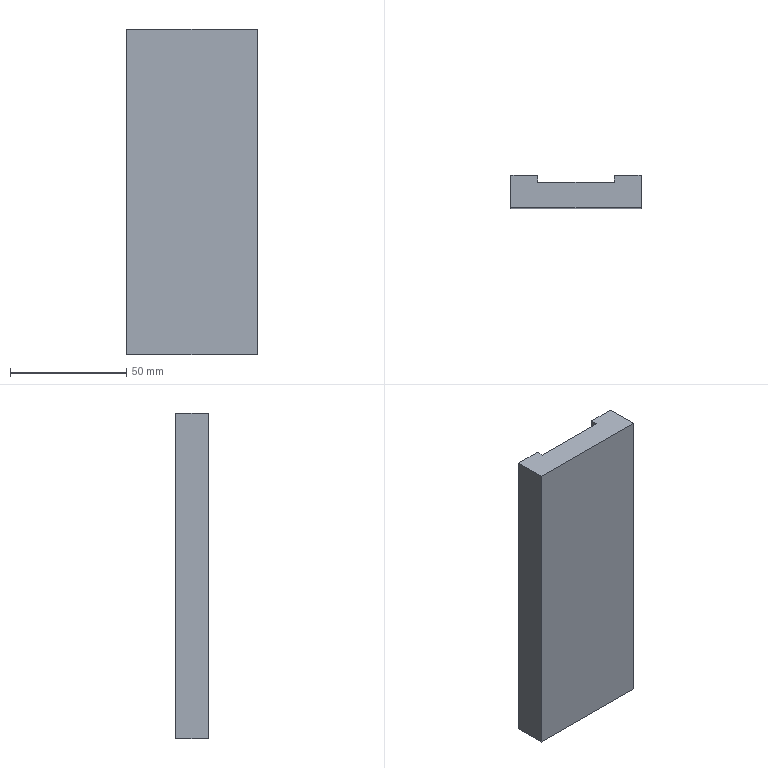Component | SolidWorks | CHEN123-AA-17-2 | 1 solid | 10 faces | box 56 x 14 x 140 mm | volume 95900 mm3 | plane 10
build123d program:
from build123d import *

# Parameters (mm, degrees)
SKETCH1_W           = 140
SKETCH1_H           = 56
BOSS_EXTRUDE1_DEPTH = 14
SKETCH3_W           = 197.23
SKETCH3_H           = 33
CUT_EXTRUDE2_DEPTH  = 3


with BuildPart() as part:
    # Sketch1 → Boss-Extrude1 (new body)
    with BuildSketch(Plane.XY):
        Rectangle(SKETCH1_W, SKETCH1_H)
    extrude(amount=BOSS_EXTRUDE1_DEPTH)

    # Sketch3 → Cut-Extrude2 (cut)
    with BuildSketch(Plane(origin=(0, 0, 0), x_dir=(-1, 0, 0), z_dir=(0, 0, -1))):
        Rectangle(SKETCH3_W, SKETCH3_H)
    extrude(amount=-CUT_EXTRUDE2_DEPTH, mode=Mode.SUBTRACT)


solid = part.part

# Placed as in the assembly
solid = solid.moved(Location((-0.0005, 34.001, -60), (90, 0, 90)))
STEP:
#1=CARTESIAN_POINT('',(-0.6496,1.339,-5.118));
#2=VERTEX_POINT('',#1);
#3=CARTESIAN_POINT('',(-0.6496,1.339,0.3937));
#4=VERTEX_POINT('',#3);
#5=CARTESIAN_POINT('',(-0.6496,1.339,-2.362));
#6=DIRECTION('',(0.,0.,1.));
#7=VECTOR('',#6,39.37);
#8=LINE('',#5,#7);
#9=EDGE_CURVE('',#2,#4,#8,.T.);
#10=ORIENTED_EDGE('',*,*,#9,.F.);
#11=CARTESIAN_POINT('',(-1.102,1.339,-5.118));
#12=VERTEX_POINT('',#11);
#13=CARTESIAN_POINT('',(1.102,1.339,-5.118));
#14=DIRECTION('',(1.,0.,-0.));
#15=VECTOR('',#14,39.37);
#16=LINE('',#13,#15);
#17=EDGE_CURVE('',#12,#2,#16,.T.);
#18=ORIENTED_EDGE('',*,*,#17,.F.);
#19=CARTESIAN_POINT('',(-1.102,1.339,0.3937));
#20=VERTEX_POINT('',#19);
#21=CARTESIAN_POINT('',(-1.102,1.339,-5.118));
#22=DIRECTION('',(-0.,0.,-1.));
#23=VECTOR('',#22,39.37);
#24=LINE('',#21,#23);
#25=EDGE_CURVE('',#20,#12,#24,.T.);
#26=ORIENTED_EDGE('',*,*,#25,.F.);
#27=CARTESIAN_POINT('',(1.102,1.339,0.3937));
#28=DIRECTION('',(-1.,0.,0.));
#29=VECTOR('',#28,39.37);
#30=LINE('',#27,#29);
#31=EDGE_CURVE('',#4,#20,#30,.T.);
#32=ORIENTED_EDGE('',*,*,#31,.F.);
#33=EDGE_LOOP('',(#10,#18,#26,#32));
#34=FACE_OUTER_BOUND('',#33,.T.);
#35=CARTESIAN_POINT('',(-0.00001969,1.339,-2.362));
#36=DIRECTION('',(0.,1.,0.));
#37=DIRECTION('',(-0.,0.,-1.));
#38=AXIS2_PLACEMENT_3D('',#35,#36,#37);
#39=PLANE('',#38);
#40=ADVANCED_FACE('',(#34),#39,.T.);
#41=CARTESIAN_POINT('',(0.6496,1.221,0.3937));
#42=VERTEX_POINT('',#41);
#43=CARTESIAN_POINT('',(-0.6496,1.221,0.3937));
#44=VERTEX_POINT('',#43);
#45=CARTESIAN_POINT('',(1.102,1.221,0.3937));
#46=DIRECTION('',(-1.,0.,0.));
#47=VECTOR('',#46,39.37);
#48=LINE('',#45,#47);
#49=EDGE_CURVE('',#42,#44,#48,.T.);
#50=ORIENTED_EDGE('',*,*,#49,.T.);
#51=CARTESIAN_POINT('',(-0.6496,0.7874,0.3937));
#52=DIRECTION('',(0.,1.,0.));
#53=VECTOR('',#52,39.37);
#54=LINE('',#51,#53);
#55=EDGE_CURVE('',#44,#4,#54,.T.);
#56=ORIENTED_EDGE('',*,*,#55,.T.);
#57=ORIENTED_EDGE('',*,*,#31,.T.);
#58=CARTESIAN_POINT('',(-1.102,0.7874,0.3937));
#59=VERTEX_POINT('',#58);
#60=CARTESIAN_POINT('',(-1.102,0.7874,0.3937));
#61=DIRECTION('',(0.,1.,0.));
#62=VECTOR('',#61,39.37);
#63=LINE('',#60,#62);
#64=EDGE_CURVE('',#59,#20,#63,.T.);
#65=ORIENTED_EDGE('',*,*,#64,.F.);
#66=CARTESIAN_POINT('',(1.102,0.7874,0.3937));
#67=VERTEX_POINT('',#66);
#68=CARTESIAN_POINT('',(1.102,0.7874,0.3937));
#69=DIRECTION('',(-1.,0.,0.));
#70=VECTOR('',#69,39.37);
#71=LINE('',#68,#70);
#72=EDGE_CURVE('',#67,#59,#71,.T.);
#73=ORIENTED_EDGE('',*,*,#72,.F.);
#74=CARTESIAN_POINT('',(1.102,1.339,0.3937));
#75=VERTEX_POINT('',#74);
#76=CARTESIAN_POINT('',(1.102,0.7874,0.3937));
#77=DIRECTION('',(0.,1.,0.));
#78=VECTOR('',#77,39.37);
#79=LINE('',#76,#78);
#80=EDGE_CURVE('',#67,#75,#79,.T.);
#81=ORIENTED_EDGE('',*,*,#80,.T.);
#82=CARTESIAN_POINT('',(0.6496,1.339,0.3937));
#83=VERTEX_POINT('',#82);
#84=CARTESIAN_POINT('',(1.102,1.339,0.3937));
#85=DIRECTION('',(-1.,0.,0.));
#86=VECTOR('',#85,39.37);
#87=LINE('',#84,#86);
#88=EDGE_CURVE('',#75,#83,#87,.T.);
#89=ORIENTED_EDGE('',*,*,#88,.T.);
#90=CARTESIAN_POINT('',(0.6496,0.7874,0.3937));
#91=DIRECTION('',(0.,-1.,0.));
#92=VECTOR('',#91,39.37);
#93=LINE('',#90,#92);
#94=EDGE_CURVE('',#83,#42,#93,.T.);
#95=ORIENTED_EDGE('',*,*,#94,.T.);
#96=EDGE_LOOP('',(#50,#56,#57,#65,#73,#81,#89,#95));
#97=FACE_OUTER_BOUND('',#96,.T.);
#98=CARTESIAN_POINT('',(1.102,0.7874,0.3937));
#99=DIRECTION('',(-0.,0.,-1.));
#100=DIRECTION('',(0.,-1.,0.));
#101=AXIS2_PLACEMENT_3D('',#98,#99,#100);
#102=PLANE('',#101);
#103=ADVANCED_FACE('',(#97),#102,.F.);
#104=ORIENTED_EDGE('',*,*,#25,.T.);
#105=CARTESIAN_POINT('',(-1.102,0.7874,-5.118));
#106=VERTEX_POINT('',#105);
#107=CARTESIAN_POINT('',(-1.102,0.7874,-5.118));
#108=DIRECTION('',(0.,1.,0.));
#109=VECTOR('',#108,39.37);
#110=LINE('',#107,#109);
#111=EDGE_CURVE('',#106,#12,#110,.T.);
#112=ORIENTED_EDGE('',*,*,#111,.F.);
#113=CARTESIAN_POINT('',(-1.102,0.7874,-5.118));
#114=DIRECTION('',(-0.,0.,-1.));
#115=VECTOR('',#114,39.37);
#116=LINE('',#113,#115);
#117=EDGE_CURVE('',#59,#106,#116,.T.);
#118=ORIENTED_EDGE('',*,*,#117,.F.);
#119=ORIENTED_EDGE('',*,*,#64,.T.);
#120=EDGE_LOOP('',(#104,#112,#118,#119));
#121=FACE_OUTER_BOUND('',#120,.T.);
#122=CARTESIAN_POINT('',(-1.102,0.7874,-5.118));
#123=DIRECTION('',(1.,0.,-0.));
#124=DIRECTION('',(0.,1.,0.));
#125=AXIS2_PLACEMENT_3D('',#122,#123,#124);
#126=PLANE('',#125);
#127=ADVANCED_FACE('',(#121),#126,.F.);
#128=ORIENTED_EDGE('',*,*,#17,.T.);
#129=CARTESIAN_POINT('',(-0.6496,1.221,-5.118));
#130=VERTEX_POINT('',#129);
#131=CARTESIAN_POINT('',(-0.6496,0.7874,-5.118));
#132=DIRECTION('',(0.,-1.,0.));
#133=VECTOR('',#132,39.37);
#134=LINE('',#131,#133);
#135=EDGE_CURVE('',#2,#130,#134,.T.);
#136=ORIENTED_EDGE('',*,*,#135,.T.);
#137=CARTESIAN_POINT('',(0.6496,1.221,-5.118));
#138=VERTEX_POINT('',#137);
#139=CARTESIAN_POINT('',(1.102,1.221,-5.118));
#140=DIRECTION('',(1.,0.,-0.));
#141=VECTOR('',#140,39.37);
#142=LINE('',#139,#141);
#143=EDGE_CURVE('',#130,#138,#142,.T.);
#144=ORIENTED_EDGE('',*,*,#143,.T.);
#145=CARTESIAN_POINT('',(0.6496,1.339,-5.118));
#146=VERTEX_POINT('',#145);
#147=CARTESIAN_POINT('',(0.6496,0.7874,-5.118));
#148=DIRECTION('',(0.,1.,0.));
#149=VECTOR('',#148,39.37);
#150=LINE('',#147,#149);
#151=EDGE_CURVE('',#138,#146,#150,.T.);
#152=ORIENTED_EDGE('',*,*,#151,.T.);
#153=CARTESIAN_POINT('',(1.102,1.339,-5.118));
#154=VERTEX_POINT('',#153);
#155=CARTESIAN_POINT('',(1.102,1.339,-5.118));
#156=DIRECTION('',(1.,0.,-0.));
#157=VECTOR('',#156,39.37);
#158=LINE('',#155,#157);
#159=EDGE_CURVE('',#146,#154,#158,.T.);
#160=ORIENTED_EDGE('',*,*,#159,.T.);
#161=CARTESIAN_POINT('',(1.102,0.7874,-5.118));
#162=VERTEX_POINT('',#161);
#163=CARTESIAN_POINT('',(1.102,0.7874,-5.118));
#164=DIRECTION('',(0.,1.,0.));
#165=VECTOR('',#164,39.37);
#166=LINE('',#163,#165);
#167=EDGE_CURVE('',#162,#154,#166,.T.);
#168=ORIENTED_EDGE('',*,*,#167,.F.);
#169=CARTESIAN_POINT('',(1.102,0.7874,-5.118));
#170=DIRECTION('',(1.,0.,-0.));
#171=VECTOR('',#170,39.37);
#172=LINE('',#169,#171);
#173=EDGE_CURVE('',#106,#162,#172,.T.);
#174=ORIENTED_EDGE('',*,*,#173,.F.);
#175=ORIENTED_EDGE('',*,*,#111,.T.);
#176=EDGE_LOOP('',(#128,#136,#144,#152,#160,#168,#174,#175));
#177=FACE_OUTER_BOUND('',#176,.T.);
#178=CARTESIAN_POINT('',(1.102,0.7874,-5.118));
#179=DIRECTION('',(0.,0.,1.));
#180=DIRECTION('',(0.,1.,0.));
#181=AXIS2_PLACEMENT_3D('',#178,#179,#180);
#182=PLANE('',#181);
#183=ADVANCED_FACE('',(#177),#182,.F.);
#184=CARTESIAN_POINT('',(1.102,1.339,-5.118));
#185=DIRECTION('',(0.,0.,1.));
#186=VECTOR('',#185,39.37);
#187=LINE('',#184,#186);
#188=EDGE_CURVE('',#154,#75,#187,.T.);
#189=ORIENTED_EDGE('',*,*,#188,.T.);
#190=ORIENTED_EDGE('',*,*,#80,.F.);
#191=CARTESIAN_POINT('',(1.102,0.7874,-5.118));
#192=DIRECTION('',(0.,0.,1.));
#193=VECTOR('',#192,39.37);
#194=LINE('',#191,#193);
#195=EDGE_CURVE('',#162,#67,#194,.T.);
#196=ORIENTED_EDGE('',*,*,#195,.F.);
#197=ORIENTED_EDGE('',*,*,#167,.T.);
#198=EDGE_LOOP('',(#189,#190,#196,#197));
#199=FACE_OUTER_BOUND('',#198,.T.);
#200=CARTESIAN_POINT('',(1.102,0.7874,-5.118));
#201=DIRECTION('',(-1.,0.,0.));
#202=DIRECTION('',(0.,-1.,0.));
#203=AXIS2_PLACEMENT_3D('',#200,#201,#202);
#204=PLANE('',#203);
#205=ADVANCED_FACE('',(#199),#204,.F.);
#206=ORIENTED_EDGE('',*,*,#72,.T.);
#207=ORIENTED_EDGE('',*,*,#117,.T.);
#208=ORIENTED_EDGE('',*,*,#173,.T.);
#209=ORIENTED_EDGE('',*,*,#195,.T.);
#210=EDGE_LOOP('',(#206,#207,#208,#209));
#211=FACE_OUTER_BOUND('',#210,.T.);
#212=CARTESIAN_POINT('',(-0.00001969,0.7874,-2.362));
#213=DIRECTION('',(0.,1.,0.));
#214=DIRECTION('',(-0.,0.,-1.));
#215=AXIS2_PLACEMENT_3D('',#212,#213,#214);
#216=PLANE('',#215);
#217=ADVANCED_FACE('',(#211),#216,.F.);
#218=CARTESIAN_POINT('',(0.6496,1.339,-2.362));
#219=DIRECTION('',(-0.,0.,-1.));
#220=VECTOR('',#219,39.37);
#221=LINE('',#218,#220);
#222=EDGE_CURVE('',#83,#146,#221,.T.);
#223=ORIENTED_EDGE('',*,*,#222,.F.);
#224=ORIENTED_EDGE('',*,*,#88,.F.);
#225=ORIENTED_EDGE('',*,*,#188,.F.);
#226=ORIENTED_EDGE('',*,*,#159,.F.);
#227=EDGE_LOOP('',(#223,#224,#225,#226));
#228=FACE_OUTER_BOUND('',#227,.T.);
#229=CARTESIAN_POINT('',(-0.00001969,1.339,-2.362));
#230=DIRECTION('',(0.,1.,0.));
#231=DIRECTION('',(-0.,0.,-1.));
#232=AXIS2_PLACEMENT_3D('',#229,#230,#231);
#233=PLANE('',#232);
#234=ADVANCED_FACE('',(#228),#233,.T.);
#235=CARTESIAN_POINT('',(0.6496,1.221,-6.245));
#236=DIRECTION('',(-0.,0.,-1.));
#237=VECTOR('',#236,39.37);
#238=LINE('',#235,#237);
#239=EDGE_CURVE('',#42,#138,#238,.T.);
#240=ORIENTED_EDGE('',*,*,#239,.T.);
#241=ORIENTED_EDGE('',*,*,#143,.F.);
#242=CARTESIAN_POINT('',(-0.6496,1.221,-6.245));
#243=DIRECTION('',(0.,0.,1.));
#244=VECTOR('',#243,39.37);
#245=LINE('',#242,#244);
#246=EDGE_CURVE('',#130,#44,#245,.T.);
#247=ORIENTED_EDGE('',*,*,#246,.T.);
#248=ORIENTED_EDGE('',*,*,#49,.F.);
#249=EDGE_LOOP('',(#240,#241,#247,#248));
#250=FACE_OUTER_BOUND('',#249,.T.);
#251=CARTESIAN_POINT('',(-0.00001969,1.221,-2.362));
#252=DIRECTION('',(0.,-1.,0.));
#253=DIRECTION('',(0.,0.,1.));
#254=AXIS2_PLACEMENT_3D('',#251,#252,#253);
#255=PLANE('',#254);
#256=ADVANCED_FACE('',(#250),#255,.F.);
#257=ORIENTED_EDGE('',*,*,#246,.F.);
#258=ORIENTED_EDGE('',*,*,#135,.F.);
#259=ORIENTED_EDGE('',*,*,#9,.T.);
#260=ORIENTED_EDGE('',*,*,#55,.F.);
#261=EDGE_LOOP('',(#257,#258,#259,#260));
#262=FACE_OUTER_BOUND('',#261,.T.);
#263=CARTESIAN_POINT('',(-0.6496,1.221,-6.245));
#264=DIRECTION('',(-1.,0.,0.));
#265=DIRECTION('',(-0.,0.,-1.));
#266=AXIS2_PLACEMENT_3D('',#263,#264,#265);
#267=PLANE('',#266);
#268=ADVANCED_FACE('',(#262),#267,.F.);
#269=ORIENTED_EDGE('',*,*,#222,.T.);
#270=ORIENTED_EDGE('',*,*,#151,.F.);
#271=ORIENTED_EDGE('',*,*,#239,.F.);
#272=ORIENTED_EDGE('',*,*,#94,.F.);
#273=EDGE_LOOP('',(#269,#270,#271,#272));
#274=FACE_OUTER_BOUND('',#273,.T.);
#275=CARTESIAN_POINT('',(0.6496,1.221,-6.245));
#276=DIRECTION('',(1.,0.,-0.));
#277=DIRECTION('',(0.,0.,1.));
#278=AXIS2_PLACEMENT_3D('',#275,#276,#277);
#279=PLANE('',#278);
#280=ADVANCED_FACE('',(#274),#279,.F.);
#281=CLOSED_SHELL('',(#40,#103,#127,#183,#205,#217,#234,#256,#268,#280));
#282=MANIFOLD_SOLID_BREP('',#281);
#283=CARTESIAN_POINT('',(0.,0.,0.));
#284=DIRECTION('',(0.,0.,1.));
#285=DIRECTION('',(1.,0.,0.));
#286=AXIS2_PLACEMENT_3D('',#283,#284,#285);
#287=(LENGTH_UNIT()NAMED_UNIT(*)SI_UNIT($,.METRE.));
#288=LENGTH_MEASURE_WITH_UNIT(LENGTH_MEASURE(0.0254),#287);
#289=DIMENSIONAL_EXPONENTS(1.,0.,0.,0.,0.,0.,0.);
#290=(CONVERSION_BASED_UNIT('',#288)LENGTH_UNIT()NAMED_UNIT(#289));
#291=UNCERTAINTY_MEASURE_WITH_UNIT(LENGTH_MEASURE(0.00001),#290,'','');
#292=(NAMED_UNIT(*)PLANE_ANGLE_UNIT()SI_UNIT($,.RADIAN.));
#293=(NAMED_UNIT(*)SI_UNIT($,.STERADIAN.)SOLID_ANGLE_UNIT());
#294=(GEOMETRIC_REPRESENTATION_CONTEXT(3)GLOBAL_UNCERTAINTY_ASSIGNED_CONTEXT((#291))GLOBAL_UNIT_ASSIGNED_CONTEXT((#290,#292,#293))REPRESENTATION_CONTEXT('',''));
#295=ADVANCED_BREP_SHAPE_REPRESENTATION('',(#282,#286),#294);
#296=COLOUR_RGB('',0.7922,0.8196,0.9333);
#297=FILL_AREA_STYLE_COLOUR('',#296);
#298=FILL_AREA_STYLE('',(#297));
#299=SURFACE_STYLE_FILL_AREA(#298);
#300=SURFACE_SIDE_STYLE('',(#299));
#301=SURFACE_STYLE_USAGE(.BOTH.,#300);
#302=PRESENTATION_STYLE_ASSIGNMENT((#301));
#303=STYLED_ITEM('',(#302),#282);
#304=PRESENTATION_LAYER_ASSIGNMENT('','',(#303));
#305=(LENGTH_UNIT()NAMED_UNIT(*)SI_UNIT($,.METRE.));
#306=LENGTH_MEASURE_WITH_UNIT(LENGTH_MEASURE(0.0254),#305);
#307=DIMENSIONAL_EXPONENTS(1.,0.,0.,0.,0.,0.,0.);
#308=(CONVERSION_BASED_UNIT('',#306)LENGTH_UNIT()NAMED_UNIT(#307));
#309=UNCERTAINTY_MEASURE_WITH_UNIT(LENGTH_MEASURE(0.00001),#308,'','');
#310=(NAMED_UNIT(*)PLANE_ANGLE_UNIT()SI_UNIT($,.RADIAN.));
#311=(NAMED_UNIT(*)SI_UNIT($,.STERADIAN.)SOLID_ANGLE_UNIT());
#312=(GEOMETRIC_REPRESENTATION_CONTEXT(3)GLOBAL_UNCERTAINTY_ASSIGNED_CONTEXT((#309))GLOBAL_UNIT_ASSIGNED_CONTEXT((#308,#310,#311))REPRESENTATION_CONTEXT('',''));
#313=MECHANICAL_DESIGN_GEOMETRIC_PRESENTATION_REPRESENTATION('',(#303),#312);